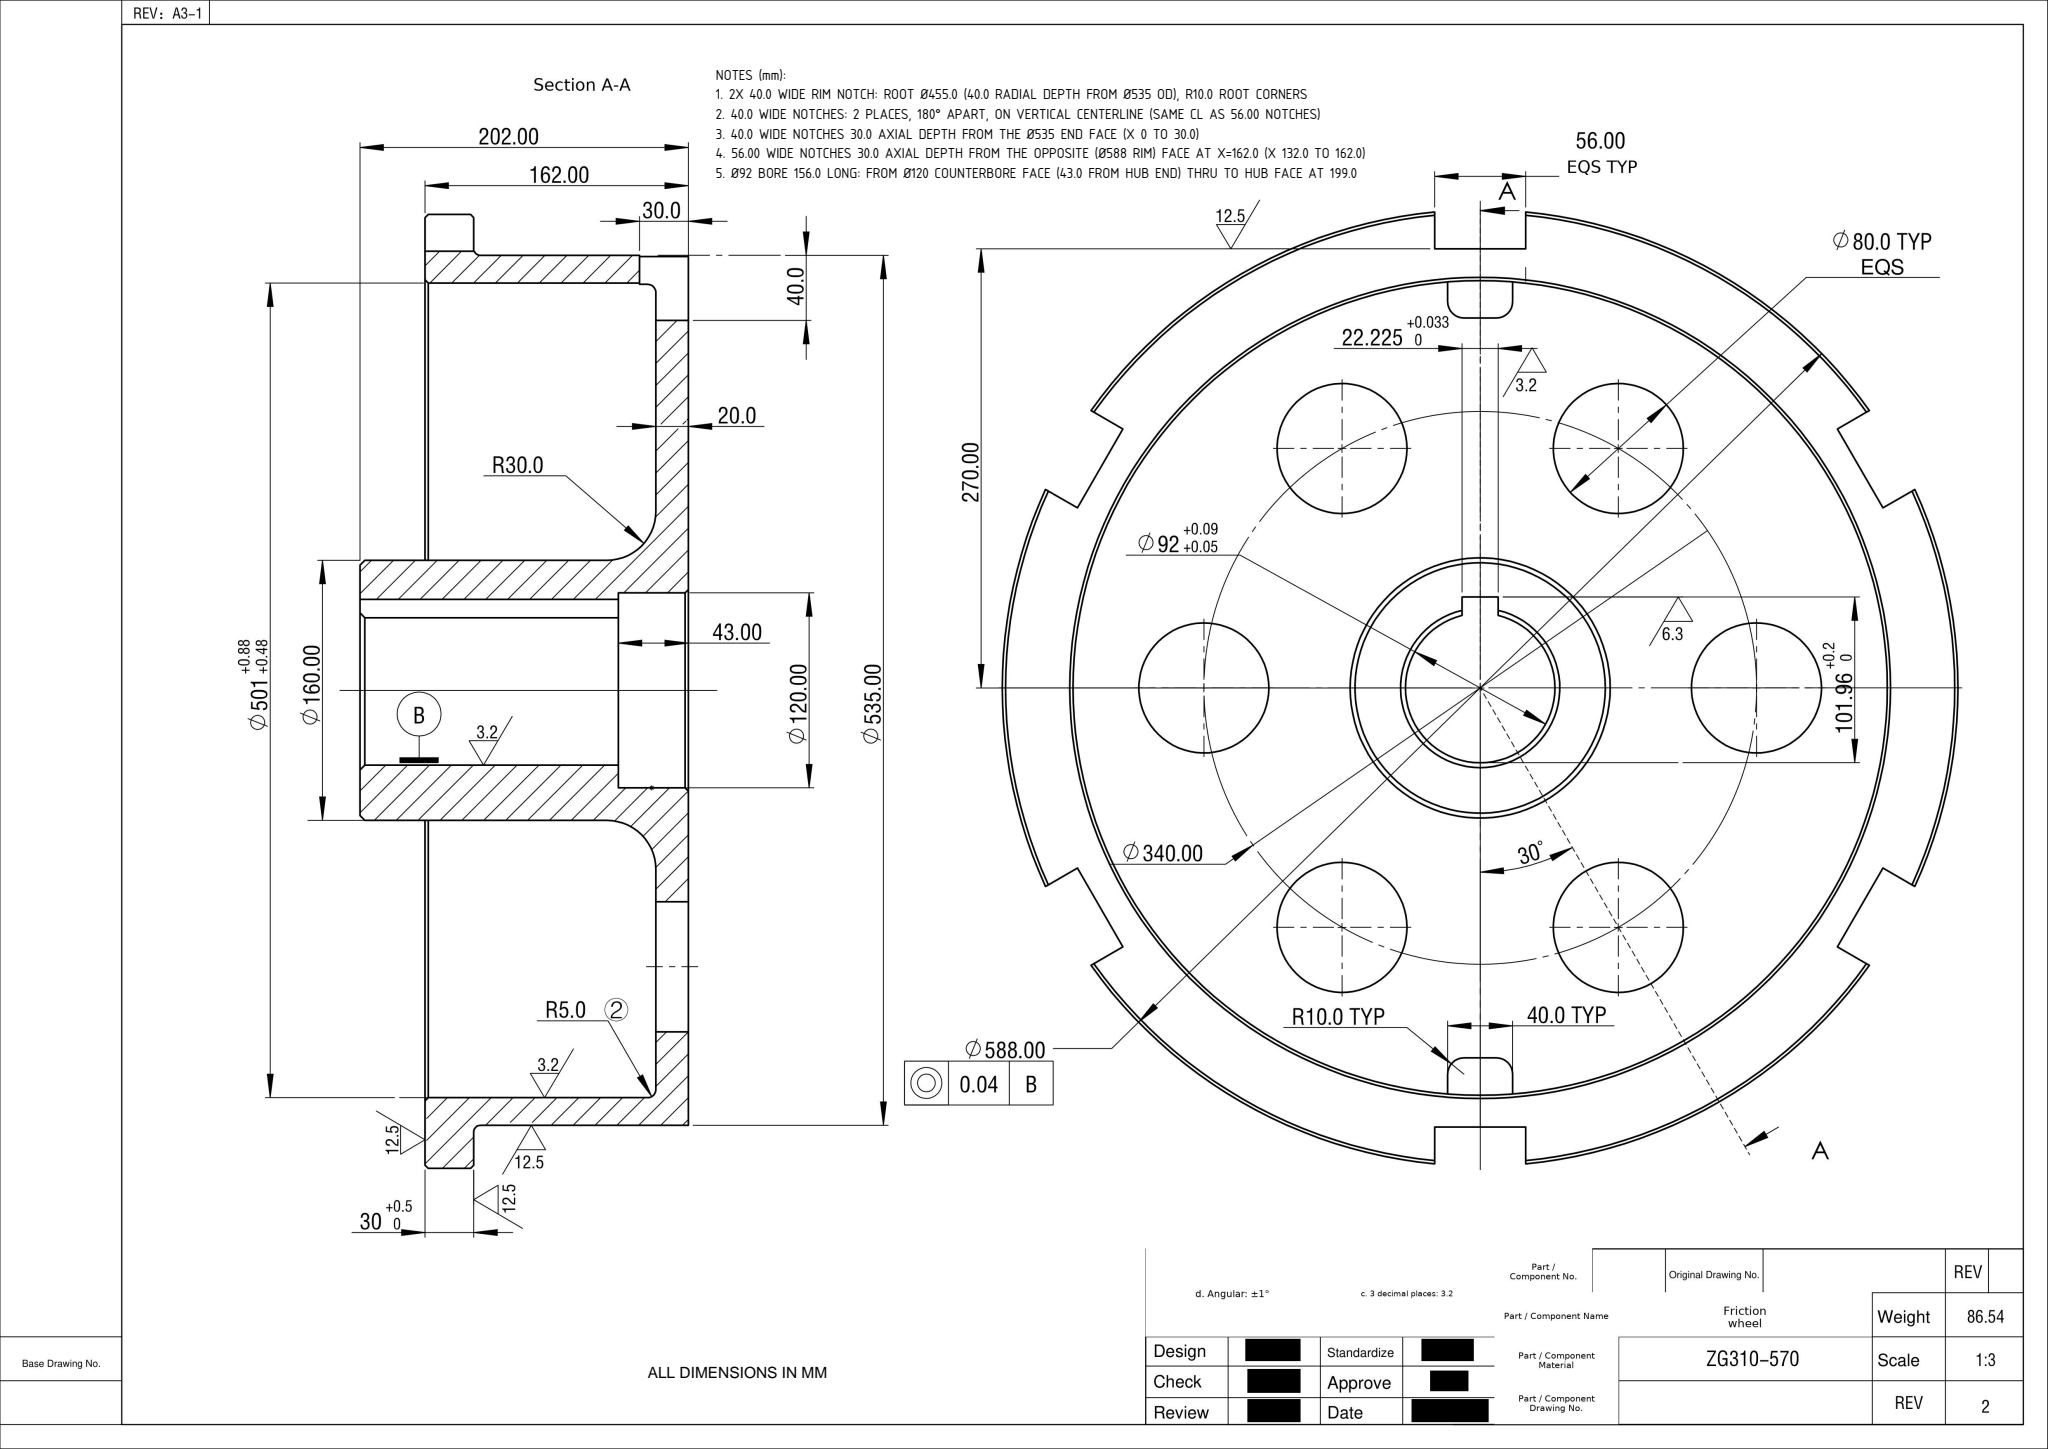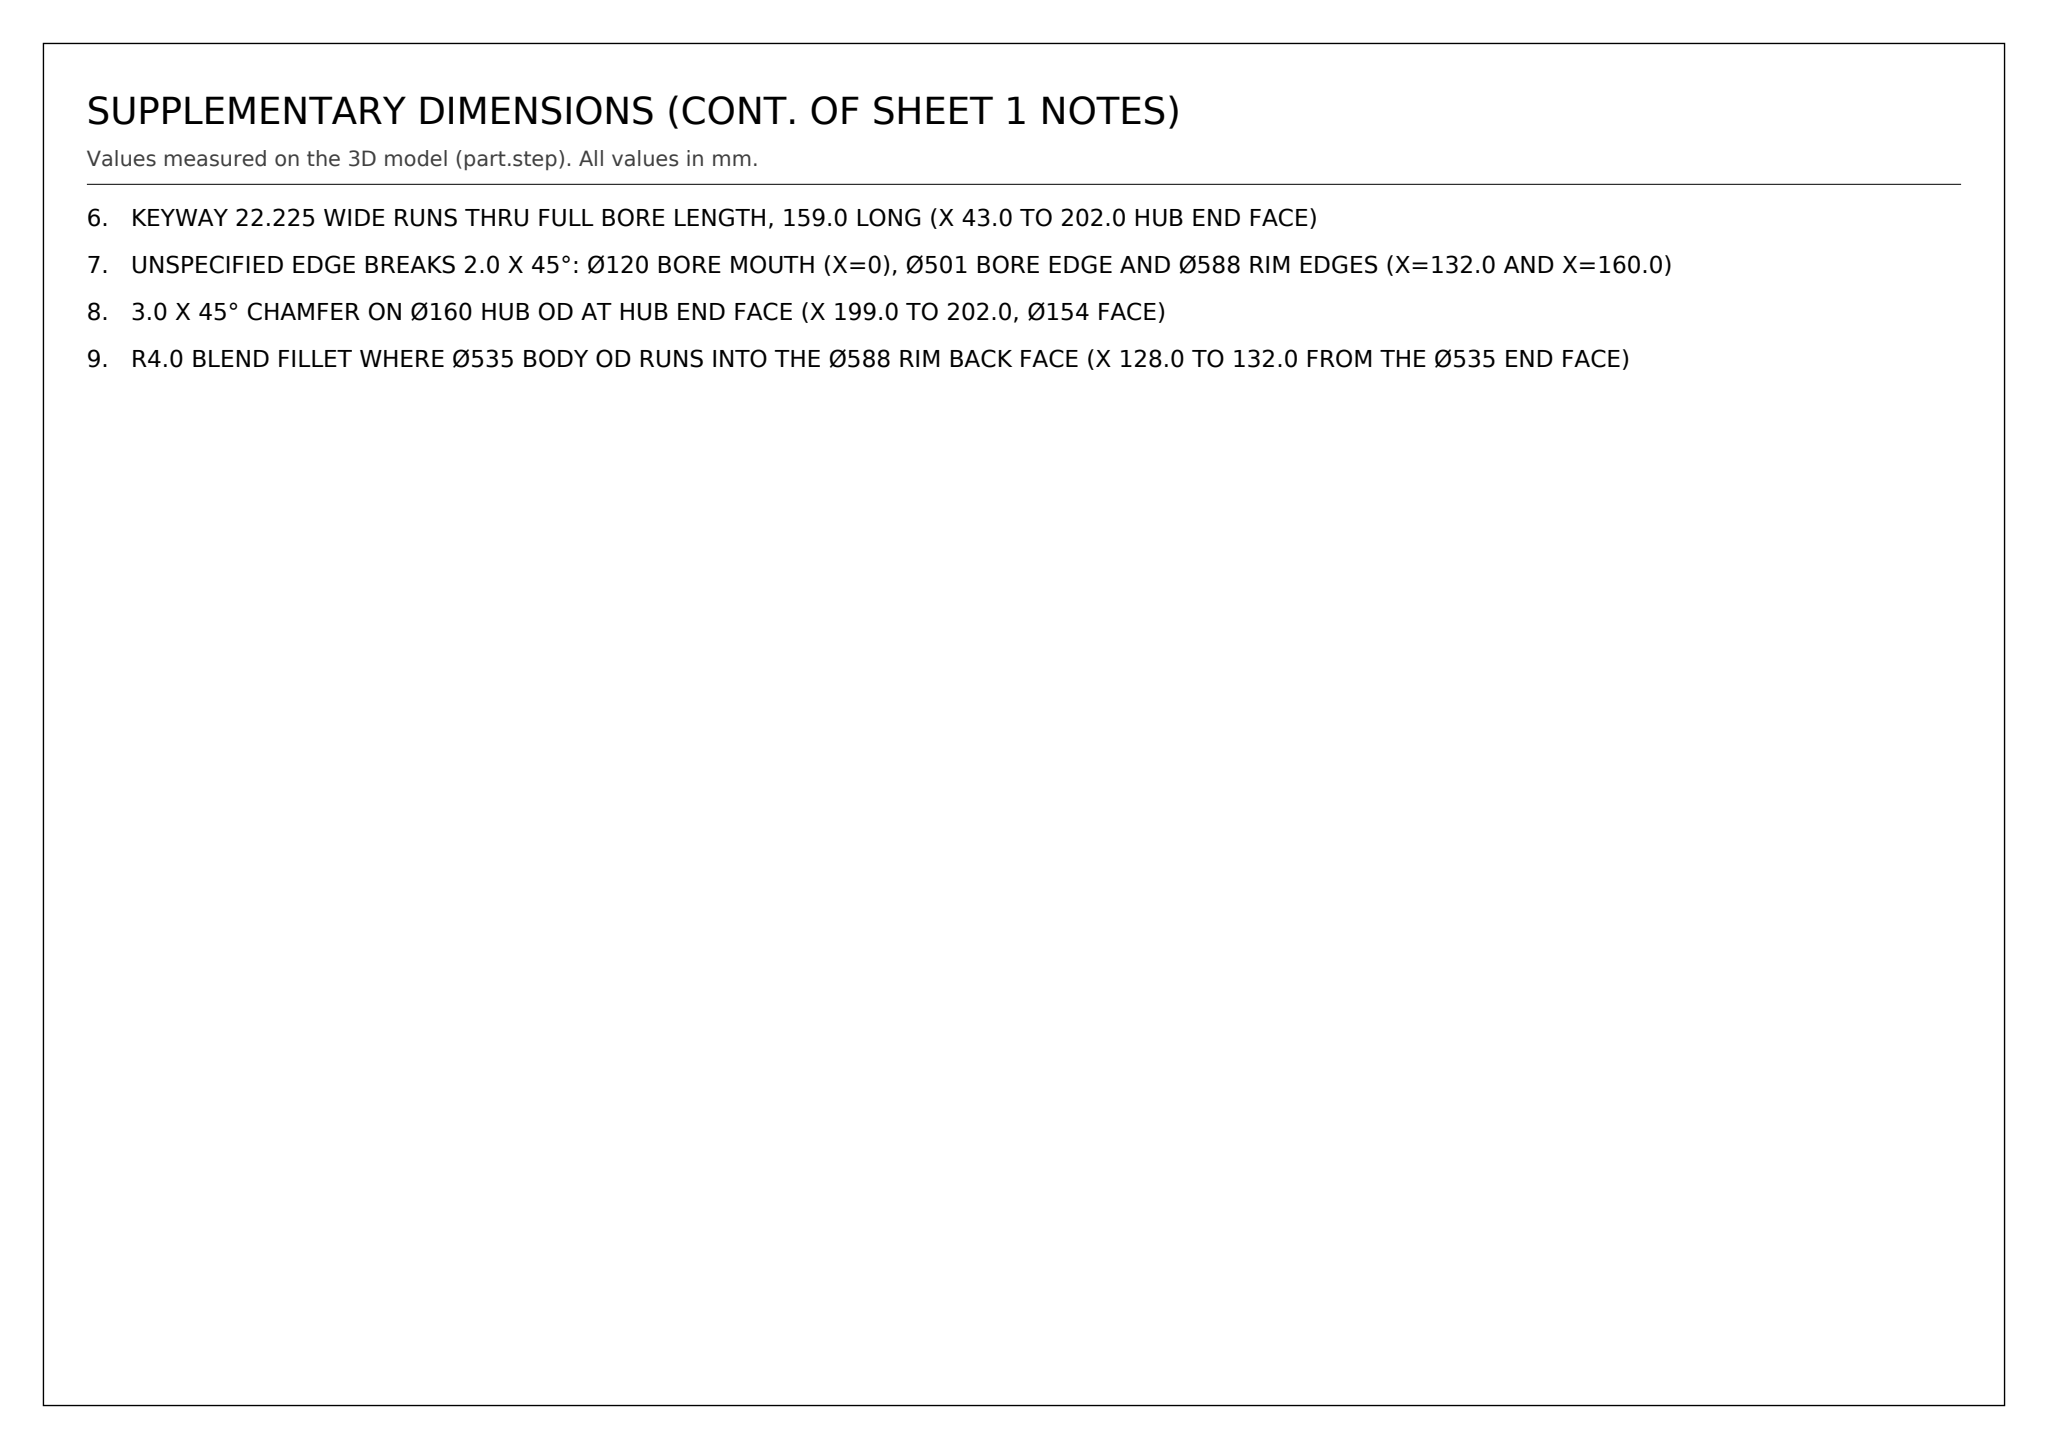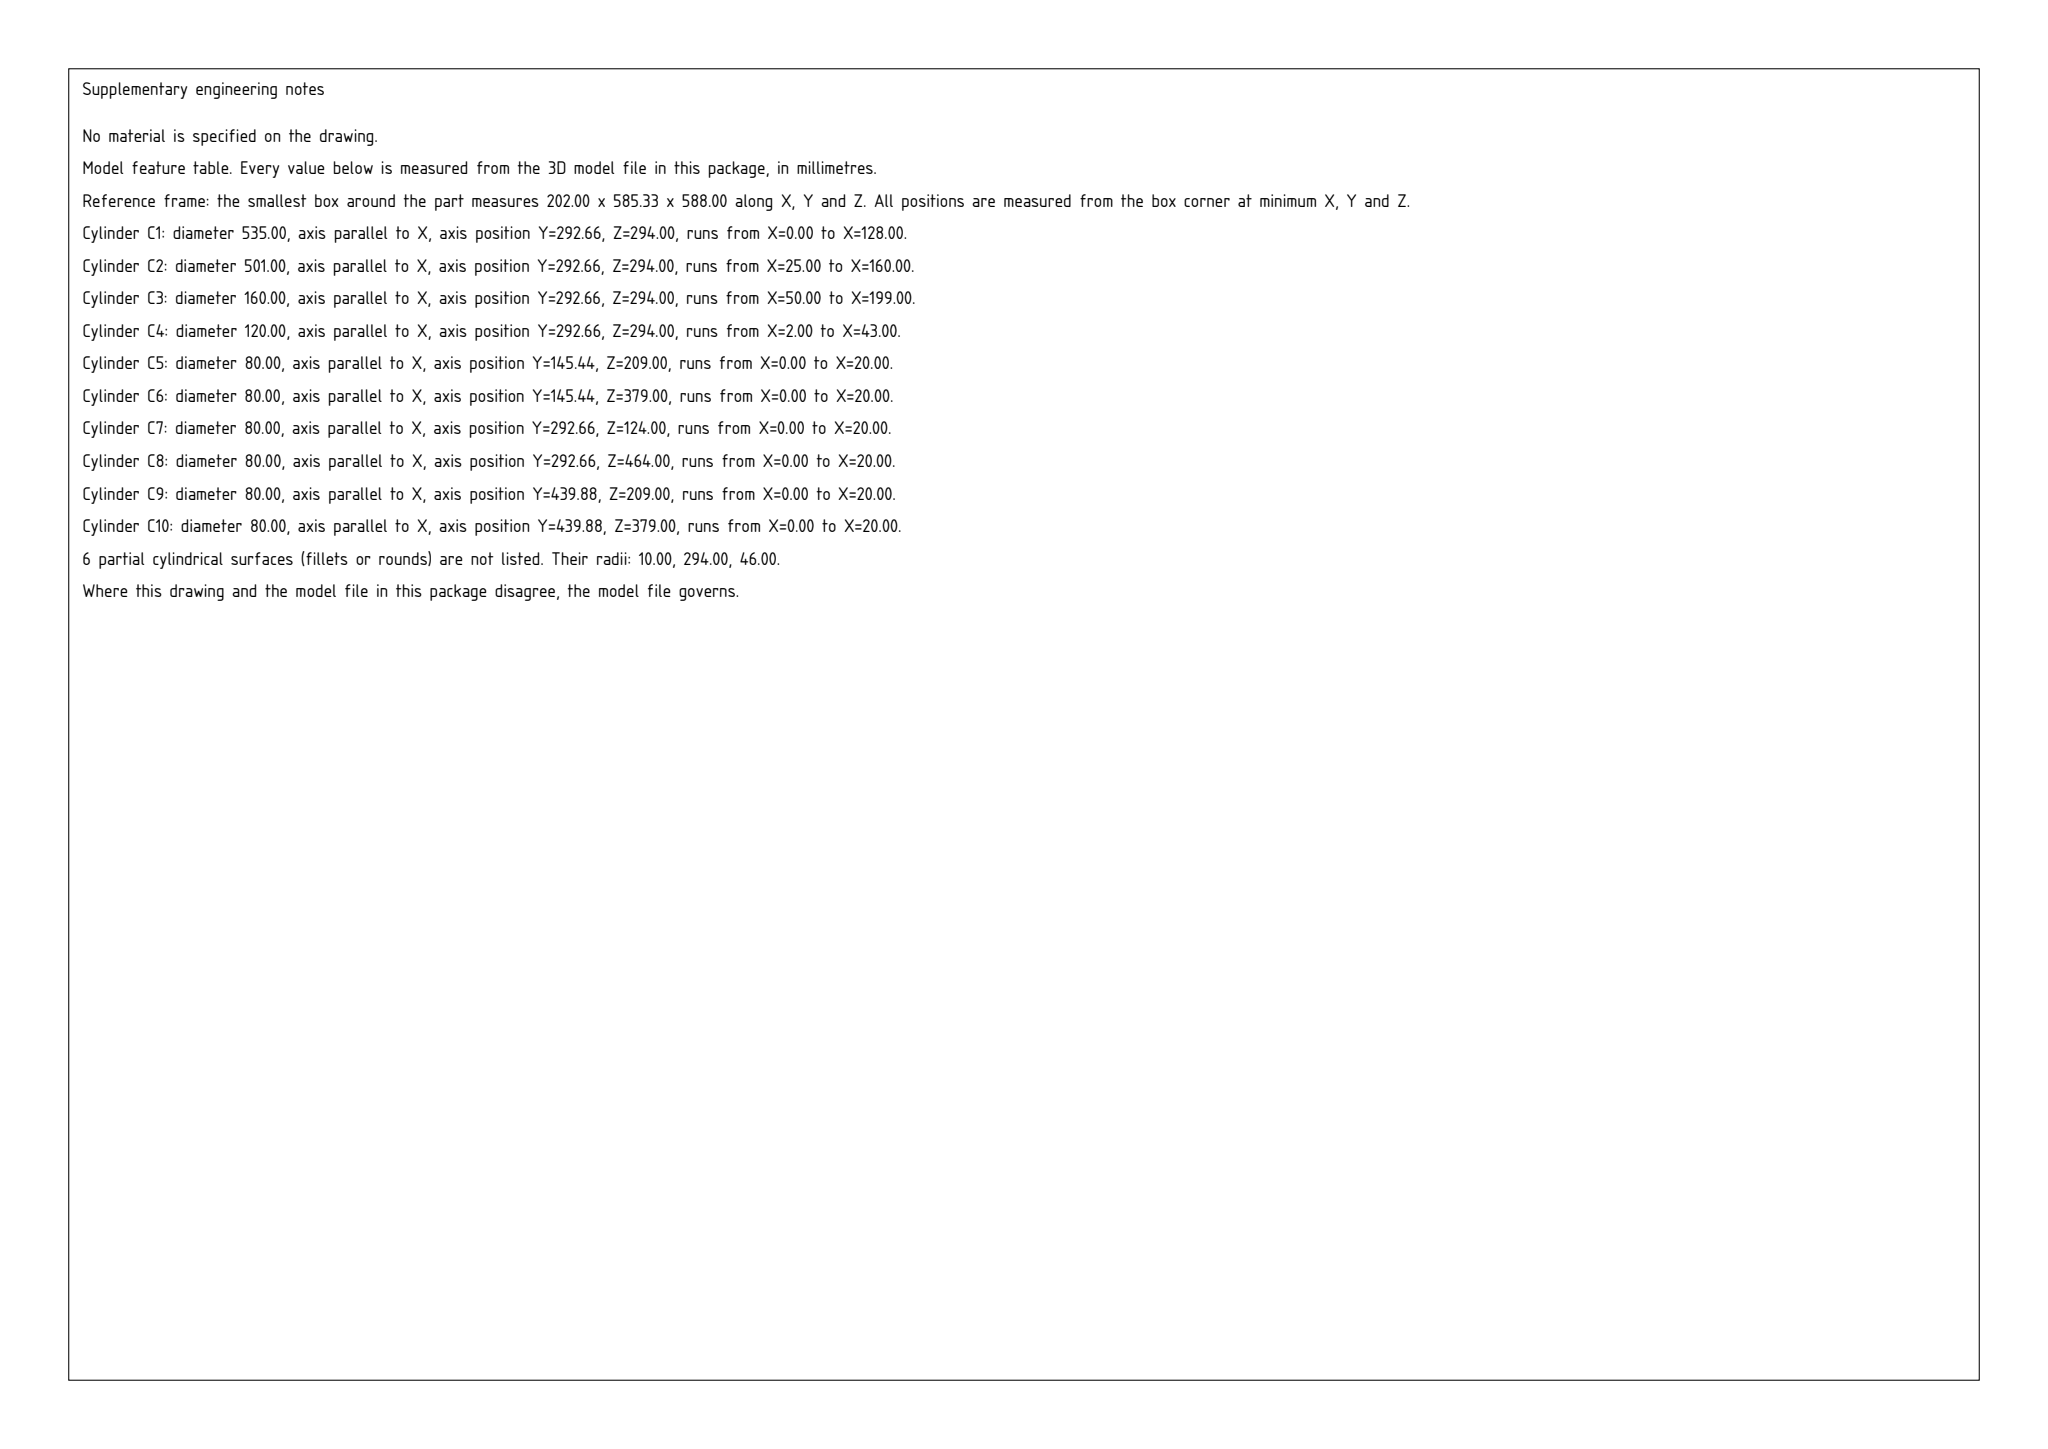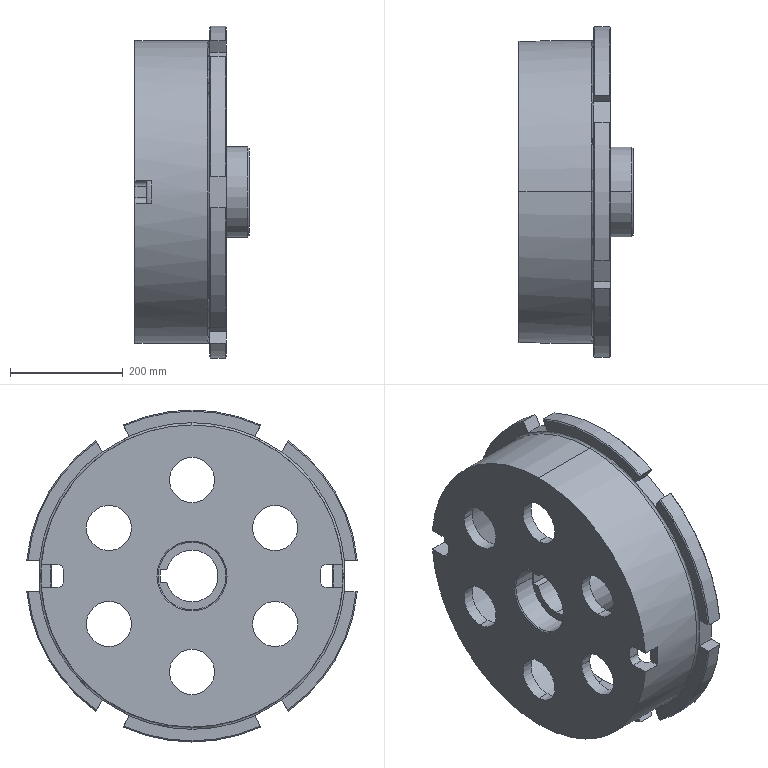Part | SolidWorks | mm | 1 solid | 104 faces | box 202 x 585.33 x 588 mm | volume 11095481 mm3 | plane 40 | cylinder 34 | cone 23 | torus 7 | commonest cylinder face diameters 80 x12 588 x7 20 x4 92 x3 120 x2 501 x2 160 x2 535 x2
Drawing notes:
2X 40.0 WIDE RIM NOTCH: ROOT Ø455.0 (40.0 RADIAL DEPTH FROM Ø535 OD), R10.0 ROOT CORNERS | from the solid: axis_planes y=69.4 and y=524.4 (z 286.9-306.9) = notch root planes, radius 296.9-69.4=227.5; concave arcs Ø20 at y=59.4/534.4
40.0 WIDE NOTCHES: 2 PLACES, 180° APART, ON VERTICAL CENTERLINE (SAME CL AS 56.00 NOTCHES) | from the solid: notch flank planes z=276.9 and z=316.9 occur only at y 30.2-59.4 and y 534.4-563.7 (two locations, y-min and y-max)
40.0 WIDE NOTCHES 30.0 AXIAL DEPTH FROM THE Ø535 END FACE (X 0 TO 30.0) | from the solid: planes z=276.9 / z=316.9 x extent [0.0, 30.0]; root plane y=69.4 x extent [0.0, 20.0]
56.00 WIDE NOTCHES 30.0 AXIAL DEPTH FROM THE OPPOSITE (Ø588 RIM) FACE AT X=162.0 (X 132.0 TO 162.0) | from the solid: axis_planes y=26.9 and y=566.9, x extent [131.7, 162.0], z 268.9-324.9 (56.0 wide) = notch root faces
Ø92 BORE 156.0 LONG: FROM Ø120 COUNTERBORE FACE (43.0 FROM HUB END) THRU TO HUB FACE AT 199.0 | from the solid: cylinder Ø92 axis x from 43.0 to 199.0; hole/bore Ø120 x from 2.0 to 43.0; plane x=43.0 (Ø120 face)
KEYWAY 22.225 WIDE RUNS THRU FULL BORE LENGTH, 159.0 LONG (X 43.0 TO 202.0 HUB END FACE) | from the solid: planes y=352.9 and z=285.8 / z=308.1, all x extent [43.0, 202.0]
UNSPECIFIED EDGE BREAKS 2.0 X 45°: Ø120 BORE MOUTH (X=0), Ø501 BORE EDGE AND Ø588 RIM EDGES (X=132.0 AND X=160.0) | from the solid: cones 90° incl.: ref dia 120 at x=0 depth 2.0; ref dia 505 at x=160 depth 2.0; ref dia 584/588 at x=132 and 160 depth 2.0
3.0 X 45° CHAMFER ON Ø160 HUB OD AT HUB END FACE (X 199.0 TO 202.0, Ø154 FACE) | from the solid: cones 90° incl. ref dia 154 at x=199.0 depth 3.0; plane x=202.0 extent 154 dia
R4.0 BLEND FILLET WHERE Ø535 BODY OD RUNS INTO THE Ø588 RIM BACK FACE (X 128.0 TO 132.0 FROM THE Ø535 END FACE) | from the solid: tori[minor_r 4.0, major_r 271.5] (=267.5 Ø535 radius + 4.0), count 2; Ø535 cylinder ends at x=128.0 and plane x=132.0 (rim back face)